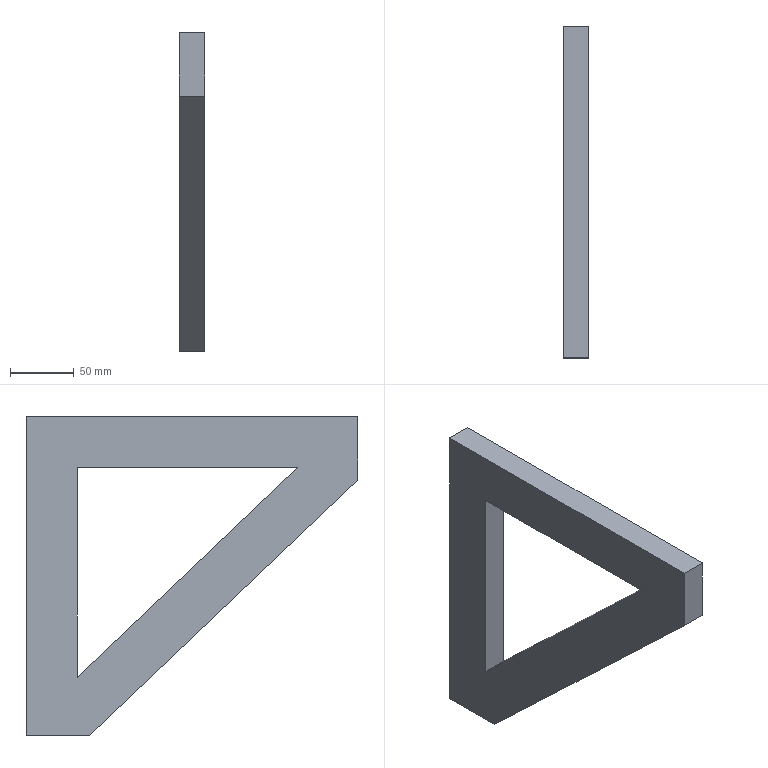Component | SolidWorks | AngleSupport-1 | 1 solid | 10 faces | box 20 x 260 x 250 mm | volume 596607 mm3 | plane 10 | material Aviation Aluminum-7075
build123d program:
from build123d import *

# Parameters (mm, degrees)
BOSS_EXTRUDE1_DEPTH = 20


with BuildPart() as part:
    # Sketch1 → Boss-Extrude1 (new body)
    with BuildSketch(Plane.XY):
        Polygon((0, 0), (-50, 0), (-260, -200), (-260, -250), (0, -250), align=None)
        Polygon((-40, -45.714), (-40, -210), (-212.5, -210), align=None, mode=Mode.SUBTRACT)
    extrude(amount=BOSS_EXTRUDE1_DEPTH)


solid = part.part

# Placed as in the assembly
solid = solid.moved(Location((115.13, -204.626, 227.215), (-90, -90, 0)))
STEP:
#1=COLOUR_RGB('',0.7922,0.8196,0.9333);
#2=FILL_AREA_STYLE_COLOUR('',#1);
#3=FILL_AREA_STYLE('',(#2));
#4=SURFACE_STYLE_FILL_AREA(#3);
#5=SURFACE_SIDE_STYLE('',(#4));
#6=SURFACE_STYLE_USAGE(.BOTH.,#5);
#7=PRESENTATION_STYLE_ASSIGNMENT((#6));
#8=CARTESIAN_POINT('',(3.745,-8.056,18.788));
#9=VERTEX_POINT('',#8);
#10=CARTESIAN_POINT('',(3.745,-8.056,8.945));
#11=VERTEX_POINT('',#10);
#12=CARTESIAN_POINT('',(3.745,-8.056,18.788));
#13=DIRECTION('',(-0.,-0.,-1.));
#14=VECTOR('',#13,39.37);
#15=LINE('',#12,#14);
#16=EDGE_CURVE('',#9,#11,#15,.T.);
#17=ORIENTED_EDGE('',*,*,#16,.T.);
#18=CARTESIAN_POINT('',(3.745,-10.025,8.945));
#19=VERTEX_POINT('',#18);
#20=CARTESIAN_POINT('',(3.745,-8.056,8.945));
#21=DIRECTION('',(-0.,-1.,0.));
#22=VECTOR('',#21,39.37);
#23=LINE('',#20,#22);
#24=EDGE_CURVE('',#11,#19,#23,.T.);
#25=ORIENTED_EDGE('',*,*,#24,.T.);
#26=CARTESIAN_POINT('',(3.745,-18.292,16.819));
#27=VERTEX_POINT('',#26);
#28=CARTESIAN_POINT('',(3.745,-10.025,8.945));
#29=DIRECTION('',(-0.,-0.7241,0.6897));
#30=VECTOR('',#29,39.37);
#31=LINE('',#28,#30);
#32=EDGE_CURVE('',#19,#27,#31,.T.);
#33=ORIENTED_EDGE('',*,*,#32,.T.);
#34=CARTESIAN_POINT('',(3.745,-18.292,18.788));
#35=VERTEX_POINT('',#34);
#36=CARTESIAN_POINT('',(3.745,-18.292,16.819));
#37=DIRECTION('',(0.,0.,1.));
#38=VECTOR('',#37,39.37);
#39=LINE('',#36,#38);
#40=EDGE_CURVE('',#27,#35,#39,.T.);
#41=ORIENTED_EDGE('',*,*,#40,.T.);
#42=CARTESIAN_POINT('',(3.745,-18.292,18.788));
#43=DIRECTION('',(0.,1.,-0.));
#44=VECTOR('',#43,39.37);
#45=LINE('',#42,#44);
#46=EDGE_CURVE('',#35,#9,#45,.T.);
#47=ORIENTED_EDGE('',*,*,#46,.T.);
#48=EDGE_LOOP('',(#17,#25,#33,#41,#47));
#49=FACE_OUTER_BOUND('',#48,.T.);
#50=CARTESIAN_POINT('',(3.745,-16.422,17.213));
#51=VERTEX_POINT('',#50);
#52=CARTESIAN_POINT('',(3.745,-9.631,17.213));
#53=VERTEX_POINT('',#52);
#54=CARTESIAN_POINT('',(3.745,-9.631,17.213));
#55=DIRECTION('',(0.,1.,-0.));
#56=VECTOR('',#55,39.37);
#57=LINE('',#54,#56);
#58=EDGE_CURVE('',#51,#53,#57,.T.);
#59=ORIENTED_EDGE('',*,*,#58,.F.);
#60=CARTESIAN_POINT('',(3.745,-9.631,10.745));
#61=VERTEX_POINT('',#60);
#62=CARTESIAN_POINT('',(3.745,-16.422,17.213));
#63=DIRECTION('',(-0.,-0.7241,0.6897));
#64=VECTOR('',#63,39.37);
#65=LINE('',#62,#64);
#66=EDGE_CURVE('',#61,#51,#65,.T.);
#67=ORIENTED_EDGE('',*,*,#66,.F.);
#68=CARTESIAN_POINT('',(3.745,-9.631,10.745));
#69=DIRECTION('',(-0.,-0.,-1.));
#70=VECTOR('',#69,39.37);
#71=LINE('',#68,#70);
#72=EDGE_CURVE('',#53,#61,#71,.T.);
#73=ORIENTED_EDGE('',*,*,#72,.F.);
#74=EDGE_LOOP('',(#59,#67,#73));
#75=FACE_BOUND('',#74,.T.);
#76=CARTESIAN_POINT('',(3.745,-8.056,8.945));
#77=DIRECTION('',(-1.,0.,0.));
#78=DIRECTION('',(0.,1.,-0.));
#79=AXIS2_PLACEMENT_3D('',#76,#77,#78);
#80=PLANE('',#79);
#81=ADVANCED_FACE('',(#49,#75),#80,.T.);
#82=CARTESIAN_POINT('',(4.533,-8.056,18.788));
#83=VERTEX_POINT('',#82);
#84=CARTESIAN_POINT('',(4.533,-8.056,8.945));
#85=VERTEX_POINT('',#84);
#86=CARTESIAN_POINT('',(4.533,-8.056,18.788));
#87=DIRECTION('',(-0.,-0.,-1.));
#88=VECTOR('',#87,39.37);
#89=LINE('',#86,#88);
#90=EDGE_CURVE('',#83,#85,#89,.T.);
#91=ORIENTED_EDGE('',*,*,#90,.F.);
#92=CARTESIAN_POINT('',(4.533,-18.292,18.788));
#93=VERTEX_POINT('',#92);
#94=CARTESIAN_POINT('',(4.533,-18.292,18.788));
#95=DIRECTION('',(0.,1.,-0.));
#96=VECTOR('',#95,39.37);
#97=LINE('',#94,#96);
#98=EDGE_CURVE('',#93,#83,#97,.T.);
#99=ORIENTED_EDGE('',*,*,#98,.F.);
#100=CARTESIAN_POINT('',(4.533,-18.292,16.819));
#101=VERTEX_POINT('',#100);
#102=CARTESIAN_POINT('',(4.533,-18.292,16.819));
#103=DIRECTION('',(0.,0.,1.));
#104=VECTOR('',#103,39.37);
#105=LINE('',#102,#104);
#106=EDGE_CURVE('',#101,#93,#105,.T.);
#107=ORIENTED_EDGE('',*,*,#106,.F.);
#108=CARTESIAN_POINT('',(4.533,-10.025,8.945));
#109=VERTEX_POINT('',#108);
#110=CARTESIAN_POINT('',(4.533,-10.025,8.945));
#111=DIRECTION('',(-0.,-0.7241,0.6897));
#112=VECTOR('',#111,39.37);
#113=LINE('',#110,#112);
#114=EDGE_CURVE('',#109,#101,#113,.T.);
#115=ORIENTED_EDGE('',*,*,#114,.F.);
#116=CARTESIAN_POINT('',(4.533,-8.056,8.945));
#117=DIRECTION('',(-0.,-1.,0.));
#118=VECTOR('',#117,39.37);
#119=LINE('',#116,#118);
#120=EDGE_CURVE('',#85,#109,#119,.T.);
#121=ORIENTED_EDGE('',*,*,#120,.F.);
#122=EDGE_LOOP('',(#91,#99,#107,#115,#121));
#123=FACE_OUTER_BOUND('',#122,.T.);
#124=CARTESIAN_POINT('',(4.533,-9.631,10.745));
#125=VERTEX_POINT('',#124);
#126=CARTESIAN_POINT('',(4.533,-16.422,17.213));
#127=VERTEX_POINT('',#126);
#128=CARTESIAN_POINT('',(4.533,-16.422,17.213));
#129=DIRECTION('',(-0.,-0.7241,0.6897));
#130=VECTOR('',#129,39.37);
#131=LINE('',#128,#130);
#132=EDGE_CURVE('',#125,#127,#131,.T.);
#133=ORIENTED_EDGE('',*,*,#132,.T.);
#134=CARTESIAN_POINT('',(4.533,-9.631,17.213));
#135=VERTEX_POINT('',#134);
#136=CARTESIAN_POINT('',(4.533,-9.631,17.213));
#137=DIRECTION('',(0.,1.,-0.));
#138=VECTOR('',#137,39.37);
#139=LINE('',#136,#138);
#140=EDGE_CURVE('',#127,#135,#139,.T.);
#141=ORIENTED_EDGE('',*,*,#140,.T.);
#142=CARTESIAN_POINT('',(4.533,-9.631,10.745));
#143=DIRECTION('',(-0.,-0.,-1.));
#144=VECTOR('',#143,39.37);
#145=LINE('',#142,#144);
#146=EDGE_CURVE('',#135,#125,#145,.T.);
#147=ORIENTED_EDGE('',*,*,#146,.T.);
#148=EDGE_LOOP('',(#133,#141,#147));
#149=FACE_BOUND('',#148,.T.);
#150=CARTESIAN_POINT('',(4.533,-8.056,8.945));
#151=DIRECTION('',(-1.,0.,0.));
#152=DIRECTION('',(0.,1.,-0.));
#153=AXIS2_PLACEMENT_3D('',#150,#151,#152);
#154=PLANE('',#153);
#155=ADVANCED_FACE('',(#123,#149),#154,.F.);
#156=ORIENTED_EDGE('',*,*,#90,.T.);
#157=CARTESIAN_POINT('',(3.745,-8.056,8.945));
#158=DIRECTION('',(1.,-0.,-0.));
#159=VECTOR('',#158,39.37);
#160=LINE('',#157,#159);
#161=EDGE_CURVE('',#11,#85,#160,.T.);
#162=ORIENTED_EDGE('',*,*,#161,.F.);
#163=ORIENTED_EDGE('',*,*,#16,.F.);
#164=CARTESIAN_POINT('',(3.745,-8.056,18.788));
#165=DIRECTION('',(1.,-0.,-0.));
#166=VECTOR('',#165,39.37);
#167=LINE('',#164,#166);
#168=EDGE_CURVE('',#9,#83,#167,.T.);
#169=ORIENTED_EDGE('',*,*,#168,.T.);
#170=EDGE_LOOP('',(#156,#162,#163,#169));
#171=FACE_OUTER_BOUND('',#170,.T.);
#172=CARTESIAN_POINT('',(3.745,-8.056,18.788));
#173=DIRECTION('',(-0.,-1.,0.));
#174=DIRECTION('',(-1.,0.,0.));
#175=AXIS2_PLACEMENT_3D('',#172,#173,#174);
#176=PLANE('',#175);
#177=ADVANCED_FACE('',(#171),#176,.F.);
#178=ORIENTED_EDGE('',*,*,#120,.T.);
#179=CARTESIAN_POINT('',(3.745,-10.025,8.945));
#180=DIRECTION('',(1.,-0.,-0.));
#181=VECTOR('',#180,39.37);
#182=LINE('',#179,#181);
#183=EDGE_CURVE('',#19,#109,#182,.T.);
#184=ORIENTED_EDGE('',*,*,#183,.F.);
#185=ORIENTED_EDGE('',*,*,#24,.F.);
#186=ORIENTED_EDGE('',*,*,#161,.T.);
#187=EDGE_LOOP('',(#178,#184,#185,#186));
#188=FACE_OUTER_BOUND('',#187,.T.);
#189=CARTESIAN_POINT('',(3.745,-8.056,8.945));
#190=DIRECTION('',(0.,0.,1.));
#191=DIRECTION('',(0.,1.,-0.));
#192=AXIS2_PLACEMENT_3D('',#189,#190,#191);
#193=PLANE('',#192);
#194=ADVANCED_FACE('',(#188),#193,.F.);
#195=ORIENTED_EDGE('',*,*,#114,.T.);
#196=CARTESIAN_POINT('',(3.745,-18.292,16.819));
#197=DIRECTION('',(1.,-0.,-0.));
#198=VECTOR('',#197,39.37);
#199=LINE('',#196,#198);
#200=EDGE_CURVE('',#27,#101,#199,.T.);
#201=ORIENTED_EDGE('',*,*,#200,.F.);
#202=ORIENTED_EDGE('',*,*,#32,.F.);
#203=ORIENTED_EDGE('',*,*,#183,.T.);
#204=EDGE_LOOP('',(#195,#201,#202,#203));
#205=FACE_OUTER_BOUND('',#204,.T.);
#206=CARTESIAN_POINT('',(3.745,-10.025,8.945));
#207=DIRECTION('',(0.,0.6897,0.7241));
#208=DIRECTION('',(0.,0.7241,-0.6897));
#209=AXIS2_PLACEMENT_3D('',#206,#207,#208);
#210=PLANE('',#209);
#211=ADVANCED_FACE('',(#205),#210,.F.);
#212=ORIENTED_EDGE('',*,*,#106,.T.);
#213=CARTESIAN_POINT('',(3.745,-18.292,18.788));
#214=DIRECTION('',(1.,-0.,-0.));
#215=VECTOR('',#214,39.37);
#216=LINE('',#213,#215);
#217=EDGE_CURVE('',#35,#93,#216,.T.);
#218=ORIENTED_EDGE('',*,*,#217,.F.);
#219=ORIENTED_EDGE('',*,*,#40,.F.);
#220=ORIENTED_EDGE('',*,*,#200,.T.);
#221=EDGE_LOOP('',(#212,#218,#219,#220));
#222=FACE_OUTER_BOUND('',#221,.T.);
#223=CARTESIAN_POINT('',(3.745,-18.292,16.819));
#224=DIRECTION('',(0.,1.,-0.));
#225=DIRECTION('',(-0.,-0.,-1.));
#226=AXIS2_PLACEMENT_3D('',#223,#224,#225);
#227=PLANE('',#226);
#228=ADVANCED_FACE('',(#222),#227,.F.);
#229=ORIENTED_EDGE('',*,*,#98,.T.);
#230=ORIENTED_EDGE('',*,*,#168,.F.);
#231=ORIENTED_EDGE('',*,*,#46,.F.);
#232=ORIENTED_EDGE('',*,*,#217,.T.);
#233=EDGE_LOOP('',(#229,#230,#231,#232));
#234=FACE_OUTER_BOUND('',#233,.T.);
#235=CARTESIAN_POINT('',(3.745,-18.292,18.788));
#236=DIRECTION('',(-0.,-0.,-1.));
#237=DIRECTION('',(-1.,0.,0.));
#238=AXIS2_PLACEMENT_3D('',#235,#236,#237);
#239=PLANE('',#238);
#240=ADVANCED_FACE('',(#234),#239,.F.);
#241=ORIENTED_EDGE('',*,*,#132,.F.);
#242=CARTESIAN_POINT('',(3.745,-9.631,10.745));
#243=DIRECTION('',(1.,-0.,-0.));
#244=VECTOR('',#243,39.37);
#245=LINE('',#242,#244);
#246=EDGE_CURVE('',#61,#125,#245,.T.);
#247=ORIENTED_EDGE('',*,*,#246,.F.);
#248=ORIENTED_EDGE('',*,*,#66,.T.);
#249=CARTESIAN_POINT('',(3.745,-16.422,17.213));
#250=DIRECTION('',(1.,-0.,-0.));
#251=VECTOR('',#250,39.37);
#252=LINE('',#249,#251);
#253=EDGE_CURVE('',#51,#127,#252,.T.);
#254=ORIENTED_EDGE('',*,*,#253,.T.);
#255=EDGE_LOOP('',(#241,#247,#248,#254));
#256=FACE_OUTER_BOUND('',#255,.T.);
#257=CARTESIAN_POINT('',(3.745,-16.422,17.213));
#258=DIRECTION('',(0.,0.6897,0.7241));
#259=DIRECTION('',(0.,0.7241,-0.6897));
#260=AXIS2_PLACEMENT_3D('',#257,#258,#259);
#261=PLANE('',#260);
#262=ADVANCED_FACE('',(#256),#261,.T.);
#263=ORIENTED_EDGE('',*,*,#140,.F.);
#264=ORIENTED_EDGE('',*,*,#253,.F.);
#265=ORIENTED_EDGE('',*,*,#58,.T.);
#266=CARTESIAN_POINT('',(3.745,-9.631,17.213));
#267=DIRECTION('',(1.,-0.,-0.));
#268=VECTOR('',#267,39.37);
#269=LINE('',#266,#268);
#270=EDGE_CURVE('',#53,#135,#269,.T.);
#271=ORIENTED_EDGE('',*,*,#270,.T.);
#272=EDGE_LOOP('',(#263,#264,#265,#271));
#273=FACE_OUTER_BOUND('',#272,.T.);
#274=CARTESIAN_POINT('',(3.745,-9.631,17.213));
#275=DIRECTION('',(-0.,-0.,-1.));
#276=DIRECTION('',(-0.,-1.,0.));
#277=AXIS2_PLACEMENT_3D('',#274,#275,#276);
#278=PLANE('',#277);
#279=ADVANCED_FACE('',(#273),#278,.T.);
#280=ORIENTED_EDGE('',*,*,#146,.F.);
#281=ORIENTED_EDGE('',*,*,#270,.F.);
#282=ORIENTED_EDGE('',*,*,#72,.T.);
#283=ORIENTED_EDGE('',*,*,#246,.T.);
#284=EDGE_LOOP('',(#280,#281,#282,#283));
#285=FACE_OUTER_BOUND('',#284,.T.);
#286=CARTESIAN_POINT('',(3.745,-9.631,10.745));
#287=DIRECTION('',(-0.,-1.,0.));
#288=DIRECTION('',(0.,0.,1.));
#289=AXIS2_PLACEMENT_3D('',#286,#287,#288);
#290=PLANE('',#289);
#291=ADVANCED_FACE('',(#285),#290,.T.);
#292=CLOSED_SHELL('',(#81,#155,#177,#194,#211,#228,#240,#262,#279,#291));
#293=MANIFOLD_SOLID_BREP('',#292);
#294=STYLED_ITEM('',(#7),#293);
#295=(LENGTH_UNIT()NAMED_UNIT(*)SI_UNIT($,.METRE.));
#296=LENGTH_MEASURE_WITH_UNIT(LENGTH_MEASURE(0.0254),#295);
#297=DIMENSIONAL_EXPONENTS(1.,0.,0.,0.,0.,0.,0.);
#298=(CONVERSION_BASED_UNIT('',#296)LENGTH_UNIT()NAMED_UNIT(#297));
#299=UNCERTAINTY_MEASURE_WITH_UNIT(LENGTH_MEASURE(0.00001),#298,'','');
#300=(NAMED_UNIT(*)PLANE_ANGLE_UNIT()SI_UNIT($,.RADIAN.));
#301=(NAMED_UNIT(*)SI_UNIT($,.STERADIAN.)SOLID_ANGLE_UNIT());
#302=(GEOMETRIC_REPRESENTATION_CONTEXT(3)GLOBAL_UNCERTAINTY_ASSIGNED_CONTEXT((#299))GLOBAL_UNIT_ASSIGNED_CONTEXT((#298,#300,#301))REPRESENTATION_CONTEXT('',''));
#303=MECHANICAL_DESIGN_GEOMETRIC_PRESENTATION_REPRESENTATION('',(#294),#302);
#304=PRESENTATION_LAYER_ASSIGNMENT('','',(#294));
#305=CARTESIAN_POINT('',(0.,0.,0.));
#306=DIRECTION('',(0.,0.,1.));
#307=DIRECTION('',(1.,0.,0.));
#308=AXIS2_PLACEMENT_3D('',#305,#306,#307);
#309=(LENGTH_UNIT()NAMED_UNIT(*)SI_UNIT($,.METRE.));
#310=LENGTH_MEASURE_WITH_UNIT(LENGTH_MEASURE(0.0254),#309);
#311=DIMENSIONAL_EXPONENTS(1.,0.,0.,0.,0.,0.,0.);
#312=(CONVERSION_BASED_UNIT('',#310)LENGTH_UNIT()NAMED_UNIT(#311));
#313=UNCERTAINTY_MEASURE_WITH_UNIT(LENGTH_MEASURE(0.00001),#312,'','');
#314=(NAMED_UNIT(*)PLANE_ANGLE_UNIT()SI_UNIT($,.RADIAN.));
#315=(NAMED_UNIT(*)SI_UNIT($,.STERADIAN.)SOLID_ANGLE_UNIT());
#316=(GEOMETRIC_REPRESENTATION_CONTEXT(3)GLOBAL_UNCERTAINTY_ASSIGNED_CONTEXT((#313))GLOBAL_UNIT_ASSIGNED_CONTEXT((#312,#314,#315))REPRESENTATION_CONTEXT('',''));
#317=ADVANCED_BREP_SHAPE_REPRESENTATION('',(#293,#308),#316);